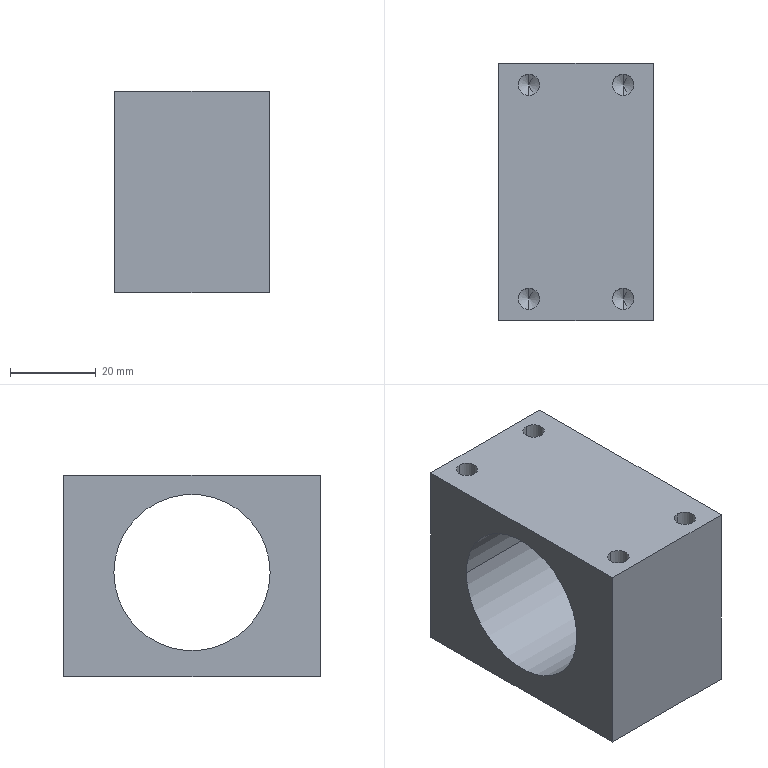Component | SolidWorks | 6G-TL06-Y-AxisMotorAssembly-2_6G-TL06.01.04-X-AxisFlangeMountingBlock-1 | 1 solid | 40 faces | box 36 x 60 x 47 mm | volume 61387 mm3 | cylinder 18 | cone 16 | plane 6 | commonest cylinder face diameters 4.2 x8 5 x8 36.5 x2
build123d program:
from build123d import *

# Parameters (mm, degrees)
SKETCH1_W             = 60
SKETCH1_H             = 36
BOSS_EXTRUDE1_DEPTH   = 47
M6_TAPPED_HOLE1_D     = 5
M6_TAPPED_HOLE1_DEPTH = 20
M6_TAPPED_HOLE1_TIP   = 1.502
M5_TAPPED_HOLE1_D     = 4.2
M5_TAPPED_HOLE1_DEPTH = 15
M5_TAPPED_HOLE1_TIP   = 1.262
SKETCH6_R             = 18.25
CUT_EXTRUDE1_DEPTH    = 67.37


with BuildPart() as part:
    # Sketch1 → Boss-Extrude1 (new body)
    with BuildSketch(Plane(origin=(0, 0, 0), x_dir=(0, 0, -1), z_dir=(1, 0, 0))):
        Rectangle(SKETCH1_W, SKETCH1_H)
    extrude(amount=BOSS_EXTRUDE1_DEPTH)

    # M6 Tapped Hole1
    with Locations(Plane(origin=(47, -3.823, -19.709), x_dir=(0, 0, 1), z_dir=(1, 0, 0))):
        with Locations((-5.291, -14.823), (-5.291, 7.177), (44.709, 7.177), (44.709, -14.823)):
            Hole(M6_TAPPED_HOLE1_D / 2, depth=M6_TAPPED_HOLE1_DEPTH)
            with Locations((0, 0, -(M6_TAPPED_HOLE1_DEPTH + M6_TAPPED_HOLE1_TIP / 2))):  # 118° drill point
                Cone(0, M6_TAPPED_HOLE1_D / 2, M6_TAPPED_HOLE1_TIP, mode=Mode.SUBTRACT)

    # M5 Tapped Hole1
    with Locations(Plane(origin=(0, -18, 0), x_dir=(-1, 0, 0), z_dir=(0, -1, 0))):
        with Locations((-40.917, -16.617), (-40.917, 16.617), (-7.683, 16.617), (-7.683, -16.617)):
            Hole(M5_TAPPED_HOLE1_D / 2, depth=M5_TAPPED_HOLE1_DEPTH)
            with Locations((0, 0, -(M5_TAPPED_HOLE1_DEPTH + M5_TAPPED_HOLE1_TIP / 2))):  # 118° drill point
                Cone(0, M5_TAPPED_HOLE1_D / 2, M5_TAPPED_HOLE1_TIP, mode=Mode.SUBTRACT)

    # Sketch6 → Cut-Extrude1 (cut, through all)
    with BuildSketch(Plane.XZ.offset(18)):
        with Locations(Location((24.3, 0, 0), (0, 0, 270))):
            Circle(SKETCH6_R)
    extrude(amount=-CUT_EXTRUDE1_DEPTH, mode=Mode.SUBTRACT)


solid = part.part

# Placed as in the assembly
solid = solid.moved(Location((-3.964, 0, -4.3), (90, 0, 90)))
STEP:
#1=CARTESIAN_POINT('',(-0.8647,-0.7185,0.7874));
#2=VERTEX_POINT('',#1);
#3=CARTESIAN_POINT('',(-0.8647,0.7185,0.7874));
#4=VERTEX_POINT('',#3);
#5=CARTESIAN_POINT('',(-0.8647,0.,0.7874));
#6=DIRECTION('',(1.,0.,-0.));
#7=DIRECTION('',(0.,1.,0.));
#8=AXIS2_PLACEMENT_3D('',#5,#6,#7);
#9=CIRCLE('',#8,0.7185);
#10=EDGE_CURVE('',#2,#4,#9,.T.);
#11=ORIENTED_EDGE('',*,*,#10,.F.);
#12=CARTESIAN_POINT('',(0.5526,-0.7185,0.7874));
#13=VERTEX_POINT('',#12);
#14=CARTESIAN_POINT('',(-0.8647,-0.7185,0.7874));
#15=DIRECTION('',(1.,0.,-0.));
#16=VECTOR('',#15,39.37);
#17=LINE('',#14,#16);
#18=EDGE_CURVE('',#2,#13,#17,.T.);
#19=ORIENTED_EDGE('',*,*,#18,.T.);
#20=CARTESIAN_POINT('',(0.5526,0.7185,0.7874));
#21=VERTEX_POINT('',#20);
#22=CARTESIAN_POINT('',(0.5526,0.,0.7874));
#23=DIRECTION('',(1.,0.,-0.));
#24=DIRECTION('',(0.,1.,0.));
#25=AXIS2_PLACEMENT_3D('',#22,#23,#24);
#26=CIRCLE('',#25,0.7185);
#27=EDGE_CURVE('',#13,#21,#26,.T.);
#28=ORIENTED_EDGE('',*,*,#27,.T.);
#29=CARTESIAN_POINT('',(-0.8647,0.7185,0.7874));
#30=DIRECTION('',(1.,0.,-0.));
#31=VECTOR('',#30,39.37);
#32=LINE('',#29,#31);
#33=EDGE_CURVE('',#4,#21,#32,.T.);
#34=ORIENTED_EDGE('',*,*,#33,.F.);
#35=EDGE_LOOP('',(#11,#19,#28,#34));
#36=FACE_OUTER_BOUND('',#35,.T.);
#37=CARTESIAN_POINT('',(-0.8647,0.,0.7874));
#38=DIRECTION('',(1.,0.,-0.));
#39=DIRECTION('',(0.,1.,0.));
#40=AXIS2_PLACEMENT_3D('',#37,#38,#39);
#41=CYLINDRICAL_SURFACE('',#40,0.7185);
#42=ADVANCED_FACE('',(#36),#41,.F.);
#43=CARTESIAN_POINT('',(-0.03795,-0.7369,1.442));
#44=VERTEX_POINT('',#43);
#45=CARTESIAN_POINT('',(-0.03795,-0.5715,1.442));
#46=VERTEX_POINT('',#45);
#47=CARTESIAN_POINT('',(-0.03795,-0.6542,1.442));
#48=DIRECTION('',(1.,0.,-0.));
#49=DIRECTION('',(0.,1.,0.));
#50=AXIS2_PLACEMENT_3D('',#47,#48,#49);
#51=CIRCLE('',#50,0.08268);
#52=EDGE_CURVE('',#44,#46,#51,.T.);
#53=ORIENTED_EDGE('',*,*,#52,.F.);
#54=CARTESIAN_POINT('',(0.5526,-0.7369,1.442));
#55=VERTEX_POINT('',#54);
#56=CARTESIAN_POINT('',(0.5526,-0.7369,1.442));
#57=DIRECTION('',(1.,0.,-0.));
#58=VECTOR('',#57,39.37);
#59=LINE('',#56,#58);
#60=EDGE_CURVE('',#44,#55,#59,.T.);
#61=ORIENTED_EDGE('',*,*,#60,.T.);
#62=CARTESIAN_POINT('',(0.5526,-0.5715,1.442));
#63=VERTEX_POINT('',#62);
#64=CARTESIAN_POINT('',(0.5526,-0.6542,1.442));
#65=DIRECTION('',(1.,0.,-0.));
#66=DIRECTION('',(0.,1.,0.));
#67=AXIS2_PLACEMENT_3D('',#64,#65,#66);
#68=CIRCLE('',#67,0.08268);
#69=EDGE_CURVE('',#55,#63,#68,.T.);
#70=ORIENTED_EDGE('',*,*,#69,.T.);
#71=CARTESIAN_POINT('',(0.5526,-0.5715,1.442));
#72=DIRECTION('',(1.,0.,-0.));
#73=VECTOR('',#72,39.37);
#74=LINE('',#71,#73);
#75=EDGE_CURVE('',#46,#63,#74,.T.);
#76=ORIENTED_EDGE('',*,*,#75,.F.);
#77=EDGE_LOOP('',(#53,#61,#70,#76));
#78=FACE_OUTER_BOUND('',#77,.T.);
#79=CARTESIAN_POINT('',(0.5526,-0.6542,1.442));
#80=DIRECTION('',(1.,0.,-0.));
#81=DIRECTION('',(0.,1.,0.));
#82=AXIS2_PLACEMENT_3D('',#79,#80,#81);
#83=CYLINDRICAL_SURFACE('',#82,0.08268);
#84=ADVANCED_FACE('',(#78),#83,.F.);
#85=CARTESIAN_POINT('',(-0.08762,-0.6542,1.442));
#86=VERTEX_POINT('',#85);
#87=CARTESIAN_POINT('',(-0.03795,-0.5715,1.442));
#88=DIRECTION('',(0.515,0.8572,0.));
#89=VECTOR('',#88,39.37);
#90=LINE('',#87,#89);
#91=EDGE_CURVE('',#86,#46,#90,.T.);
#92=ORIENTED_EDGE('',*,*,#91,.F.);
#93=CARTESIAN_POINT('',(-0.03795,-0.7369,1.442));
#94=DIRECTION('',(0.515,-0.8572,-0.));
#95=VECTOR('',#94,39.37);
#96=LINE('',#93,#95);
#97=EDGE_CURVE('',#86,#44,#96,.T.);
#98=ORIENTED_EDGE('',*,*,#97,.T.);
#99=ORIENTED_EDGE('',*,*,#52,.T.);
#100=EDGE_LOOP('',(#92,#98,#99));
#101=FACE_OUTER_BOUND('',#100,.T.);
#102=CARTESIAN_POINT('',(-0.03795,-0.6542,1.442));
#103=DIRECTION('',(1.,0.,-0.));
#104=DIRECTION('',(0.,1.,0.));
#105=AXIS2_PLACEMENT_3D('',#102,#103,#104);
#106=CONICAL_SURFACE('',#105,0.08268,1.03);
#107=ADVANCED_FACE('',(#101),#106,.F.);
#108=CARTESIAN_POINT('',(-0.03795,0.5715,1.442));
#109=VERTEX_POINT('',#108);
#110=CARTESIAN_POINT('',(-0.03795,0.7369,1.442));
#111=VERTEX_POINT('',#110);
#112=CARTESIAN_POINT('',(-0.03795,0.6542,1.442));
#113=DIRECTION('',(1.,0.,-0.));
#114=DIRECTION('',(0.,1.,0.));
#115=AXIS2_PLACEMENT_3D('',#112,#113,#114);
#116=CIRCLE('',#115,0.08268);
#117=EDGE_CURVE('',#109,#111,#116,.T.);
#118=ORIENTED_EDGE('',*,*,#117,.F.);
#119=CARTESIAN_POINT('',(0.5526,0.5715,1.442));
#120=VERTEX_POINT('',#119);
#121=CARTESIAN_POINT('',(0.5526,0.5715,1.442));
#122=DIRECTION('',(1.,0.,-0.));
#123=VECTOR('',#122,39.37);
#124=LINE('',#121,#123);
#125=EDGE_CURVE('',#109,#120,#124,.T.);
#126=ORIENTED_EDGE('',*,*,#125,.T.);
#127=CARTESIAN_POINT('',(0.5526,0.7369,1.442));
#128=VERTEX_POINT('',#127);
#129=CARTESIAN_POINT('',(0.5526,0.6542,1.442));
#130=DIRECTION('',(1.,0.,-0.));
#131=DIRECTION('',(0.,1.,0.));
#132=AXIS2_PLACEMENT_3D('',#129,#130,#131);
#133=CIRCLE('',#132,0.08268);
#134=EDGE_CURVE('',#120,#128,#133,.T.);
#135=ORIENTED_EDGE('',*,*,#134,.T.);
#136=CARTESIAN_POINT('',(0.5526,0.7369,1.442));
#137=DIRECTION('',(1.,0.,-0.));
#138=VECTOR('',#137,39.37);
#139=LINE('',#136,#138);
#140=EDGE_CURVE('',#111,#128,#139,.T.);
#141=ORIENTED_EDGE('',*,*,#140,.F.);
#142=EDGE_LOOP('',(#118,#126,#135,#141));
#143=FACE_OUTER_BOUND('',#142,.T.);
#144=CARTESIAN_POINT('',(0.5526,0.6542,1.442));
#145=DIRECTION('',(1.,0.,-0.));
#146=DIRECTION('',(0.,1.,0.));
#147=AXIS2_PLACEMENT_3D('',#144,#145,#146);
#148=CYLINDRICAL_SURFACE('',#147,0.08268);
#149=ADVANCED_FACE('',(#143),#148,.F.);
#150=CARTESIAN_POINT('',(-0.08762,0.6542,1.442));
#151=VERTEX_POINT('',#150);
#152=CARTESIAN_POINT('',(-0.03795,0.7369,1.442));
#153=DIRECTION('',(0.515,0.8572,0.));
#154=VECTOR('',#153,39.37);
#155=LINE('',#152,#154);
#156=EDGE_CURVE('',#151,#111,#155,.T.);
#157=ORIENTED_EDGE('',*,*,#156,.F.);
#158=CARTESIAN_POINT('',(-0.03795,0.5715,1.442));
#159=DIRECTION('',(0.515,-0.8572,-0.));
#160=VECTOR('',#159,39.37);
#161=LINE('',#158,#160);
#162=EDGE_CURVE('',#151,#109,#161,.T.);
#163=ORIENTED_EDGE('',*,*,#162,.T.);
#164=ORIENTED_EDGE('',*,*,#117,.T.);
#165=EDGE_LOOP('',(#157,#163,#164));
#166=FACE_OUTER_BOUND('',#165,.T.);
#167=CARTESIAN_POINT('',(-0.03795,0.6542,1.442));
#168=DIRECTION('',(1.,0.,-0.));
#169=DIRECTION('',(0.,1.,0.));
#170=AXIS2_PLACEMENT_3D('',#167,#168,#169);
#171=CONICAL_SURFACE('',#170,0.08268,1.03);
#172=ADVANCED_FACE('',(#166),#171,.F.);
#173=CARTESIAN_POINT('',(-0.03795,0.5715,0.1332));
#174=VERTEX_POINT('',#173);
#175=CARTESIAN_POINT('',(-0.03795,0.7369,0.1332));
#176=VERTEX_POINT('',#175);
#177=CARTESIAN_POINT('',(-0.03795,0.6542,0.1332));
#178=DIRECTION('',(1.,0.,-0.));
#179=DIRECTION('',(0.,1.,0.));
#180=AXIS2_PLACEMENT_3D('',#177,#178,#179);
#181=CIRCLE('',#180,0.08268);
#182=EDGE_CURVE('',#174,#176,#181,.T.);
#183=ORIENTED_EDGE('',*,*,#182,.F.);
#184=CARTESIAN_POINT('',(0.5526,0.5715,0.1332));
#185=VERTEX_POINT('',#184);
#186=CARTESIAN_POINT('',(0.5526,0.5715,0.1332));
#187=DIRECTION('',(1.,0.,-0.));
#188=VECTOR('',#187,39.37);
#189=LINE('',#186,#188);
#190=EDGE_CURVE('',#174,#185,#189,.T.);
#191=ORIENTED_EDGE('',*,*,#190,.T.);
#192=CARTESIAN_POINT('',(0.5526,0.7369,0.1332));
#193=VERTEX_POINT('',#192);
#194=CARTESIAN_POINT('',(0.5526,0.6542,0.1332));
#195=DIRECTION('',(1.,0.,-0.));
#196=DIRECTION('',(0.,1.,0.));
#197=AXIS2_PLACEMENT_3D('',#194,#195,#196);
#198=CIRCLE('',#197,0.08268);
#199=EDGE_CURVE('',#185,#193,#198,.T.);
#200=ORIENTED_EDGE('',*,*,#199,.T.);
#201=CARTESIAN_POINT('',(0.5526,0.7369,0.1332));
#202=DIRECTION('',(1.,0.,-0.));
#203=VECTOR('',#202,39.37);
#204=LINE('',#201,#203);
#205=EDGE_CURVE('',#176,#193,#204,.T.);
#206=ORIENTED_EDGE('',*,*,#205,.F.);
#207=EDGE_LOOP('',(#183,#191,#200,#206));
#208=FACE_OUTER_BOUND('',#207,.T.);
#209=CARTESIAN_POINT('',(0.5526,0.6542,0.1332));
#210=DIRECTION('',(1.,0.,-0.));
#211=DIRECTION('',(0.,1.,0.));
#212=AXIS2_PLACEMENT_3D('',#209,#210,#211);
#213=CYLINDRICAL_SURFACE('',#212,0.08268);
#214=ADVANCED_FACE('',(#208),#213,.F.);
#215=CARTESIAN_POINT('',(-0.08762,0.6542,0.1332));
#216=VERTEX_POINT('',#215);
#217=CARTESIAN_POINT('',(-0.03795,0.7369,0.1332));
#218=DIRECTION('',(0.515,0.8572,0.));
#219=VECTOR('',#218,39.37);
#220=LINE('',#217,#219);
#221=EDGE_CURVE('',#216,#176,#220,.T.);
#222=ORIENTED_EDGE('',*,*,#221,.F.);
#223=CARTESIAN_POINT('',(-0.03795,0.5715,0.1332));
#224=DIRECTION('',(0.515,-0.8572,-0.));
#225=VECTOR('',#224,39.37);
#226=LINE('',#223,#225);
#227=EDGE_CURVE('',#216,#174,#226,.T.);
#228=ORIENTED_EDGE('',*,*,#227,.T.);
#229=ORIENTED_EDGE('',*,*,#182,.T.);
#230=EDGE_LOOP('',(#222,#228,#229));
#231=FACE_OUTER_BOUND('',#230,.T.);
#232=CARTESIAN_POINT('',(-0.03795,0.6542,0.1332));
#233=DIRECTION('',(1.,0.,-0.));
#234=DIRECTION('',(0.,1.,0.));
#235=AXIS2_PLACEMENT_3D('',#232,#233,#234);
#236=CONICAL_SURFACE('',#235,0.08268,1.03);
#237=ADVANCED_FACE('',(#231),#236,.F.);
#238=CARTESIAN_POINT('',(-0.03795,-0.7369,0.1332));
#239=VERTEX_POINT('',#238);
#240=CARTESIAN_POINT('',(-0.03795,-0.5715,0.1332));
#241=VERTEX_POINT('',#240);
#242=CARTESIAN_POINT('',(-0.03795,-0.6542,0.1332));
#243=DIRECTION('',(1.,0.,-0.));
#244=DIRECTION('',(0.,1.,0.));
#245=AXIS2_PLACEMENT_3D('',#242,#243,#244);
#246=CIRCLE('',#245,0.08268);
#247=EDGE_CURVE('',#239,#241,#246,.T.);
#248=ORIENTED_EDGE('',*,*,#247,.F.);
#249=CARTESIAN_POINT('',(0.5526,-0.7369,0.1332));
#250=VERTEX_POINT('',#249);
#251=CARTESIAN_POINT('',(0.5526,-0.7369,0.1332));
#252=DIRECTION('',(1.,0.,-0.));
#253=VECTOR('',#252,39.37);
#254=LINE('',#251,#253);
#255=EDGE_CURVE('',#239,#250,#254,.T.);
#256=ORIENTED_EDGE('',*,*,#255,.T.);
#257=CARTESIAN_POINT('',(0.5526,-0.5715,0.1332));
#258=VERTEX_POINT('',#257);
#259=CARTESIAN_POINT('',(0.5526,-0.6542,0.1332));
#260=DIRECTION('',(1.,0.,-0.));
#261=DIRECTION('',(0.,1.,0.));
#262=AXIS2_PLACEMENT_3D('',#259,#260,#261);
#263=CIRCLE('',#262,0.08268);
#264=EDGE_CURVE('',#250,#258,#263,.T.);
#265=ORIENTED_EDGE('',*,*,#264,.T.);
#266=CARTESIAN_POINT('',(0.5526,-0.5715,0.1332));
#267=DIRECTION('',(1.,0.,-0.));
#268=VECTOR('',#267,39.37);
#269=LINE('',#266,#268);
#270=EDGE_CURVE('',#241,#258,#269,.T.);
#271=ORIENTED_EDGE('',*,*,#270,.F.);
#272=EDGE_LOOP('',(#248,#256,#265,#271));
#273=FACE_OUTER_BOUND('',#272,.T.);
#274=CARTESIAN_POINT('',(0.5526,-0.6542,0.1332));
#275=DIRECTION('',(1.,0.,-0.));
#276=DIRECTION('',(0.,1.,0.));
#277=AXIS2_PLACEMENT_3D('',#274,#275,#276);
#278=CYLINDRICAL_SURFACE('',#277,0.08268);
#279=ADVANCED_FACE('',(#273),#278,.F.);
#280=CARTESIAN_POINT('',(-0.08762,-0.6542,0.1332));
#281=VERTEX_POINT('',#280);
#282=CARTESIAN_POINT('',(-0.03795,-0.5715,0.1332));
#283=DIRECTION('',(0.515,0.8572,0.));
#284=VECTOR('',#283,39.37);
#285=LINE('',#282,#284);
#286=EDGE_CURVE('',#281,#241,#285,.T.);
#287=ORIENTED_EDGE('',*,*,#286,.F.);
#288=CARTESIAN_POINT('',(-0.03795,-0.7369,0.1332));
#289=DIRECTION('',(0.515,-0.8572,-0.));
#290=VECTOR('',#289,39.37);
#291=LINE('',#288,#290);
#292=EDGE_CURVE('',#281,#239,#291,.T.);
#293=ORIENTED_EDGE('',*,*,#292,.T.);
#294=ORIENTED_EDGE('',*,*,#247,.T.);
#295=EDGE_LOOP('',(#287,#293,#294));
#296=FACE_OUTER_BOUND('',#295,.T.);
#297=CARTESIAN_POINT('',(-0.03795,-0.6542,0.1332));
#298=DIRECTION('',(1.,0.,-0.));
#299=DIRECTION('',(0.,1.,0.));
#300=AXIS2_PLACEMENT_3D('',#297,#298,#299);
#301=CONICAL_SURFACE('',#300,0.08268,1.03);
#302=ADVANCED_FACE('',(#296),#301,.F.);
#303=CARTESIAN_POINT('',(-0.5891,0.8858,0.8937));
#304=VERTEX_POINT('',#303);
#305=CARTESIAN_POINT('',(-0.5891,1.083,0.8937));
#306=VERTEX_POINT('',#305);
#307=CARTESIAN_POINT('',(-0.5891,0.9843,0.8937));
#308=DIRECTION('',(0.,-0.,1.));
#309=DIRECTION('',(0.,1.,0.));
#310=AXIS2_PLACEMENT_3D('',#307,#308,#309);
#311=CIRCLE('',#310,0.09843);
#312=EDGE_CURVE('',#304,#306,#311,.T.);
#313=ORIENTED_EDGE('',*,*,#312,.F.);
#314=CARTESIAN_POINT('',(-0.5891,0.8858,1.681));
#315=VERTEX_POINT('',#314);
#316=CARTESIAN_POINT('',(-0.5891,0.8858,1.681));
#317=DIRECTION('',(0.,-0.,1.));
#318=VECTOR('',#317,39.37);
#319=LINE('',#316,#318);
#320=EDGE_CURVE('',#304,#315,#319,.T.);
#321=ORIENTED_EDGE('',*,*,#320,.T.);
#322=CARTESIAN_POINT('',(-0.5891,1.083,1.681));
#323=VERTEX_POINT('',#322);
#324=CARTESIAN_POINT('',(-0.5891,0.9843,1.681));
#325=DIRECTION('',(0.,-0.,1.));
#326=DIRECTION('',(0.,1.,0.));
#327=AXIS2_PLACEMENT_3D('',#324,#325,#326);
#328=CIRCLE('',#327,0.09843);
#329=EDGE_CURVE('',#315,#323,#328,.T.);
#330=ORIENTED_EDGE('',*,*,#329,.T.);
#331=CARTESIAN_POINT('',(-0.5891,1.083,1.681));
#332=DIRECTION('',(0.,-0.,1.));
#333=VECTOR('',#332,39.37);
#334=LINE('',#331,#333);
#335=EDGE_CURVE('',#306,#323,#334,.T.);
#336=ORIENTED_EDGE('',*,*,#335,.F.);
#337=EDGE_LOOP('',(#313,#321,#330,#336));
#338=FACE_OUTER_BOUND('',#337,.T.);
#339=CARTESIAN_POINT('',(-0.5891,0.9843,1.681));
#340=DIRECTION('',(0.,-0.,1.));
#341=DIRECTION('',(0.,1.,0.));
#342=AXIS2_PLACEMENT_3D('',#339,#340,#341);
#343=CYLINDRICAL_SURFACE('',#342,0.09843);
#344=ADVANCED_FACE('',(#338),#343,.F.);
#345=CARTESIAN_POINT('',(-0.5891,0.9843,0.8346));
#346=VERTEX_POINT('',#345);
#347=CARTESIAN_POINT('',(-0.5891,1.083,0.8937));
#348=DIRECTION('',(-0.,0.8572,0.515));
#349=VECTOR('',#348,39.37);
#350=LINE('',#347,#349);
#351=EDGE_CURVE('',#346,#306,#350,.T.);
#352=ORIENTED_EDGE('',*,*,#351,.F.);
#353=CARTESIAN_POINT('',(-0.5891,0.8858,0.8937));
#354=DIRECTION('',(-0.,-0.8572,0.515));
#355=VECTOR('',#354,39.37);
#356=LINE('',#353,#355);
#357=EDGE_CURVE('',#346,#304,#356,.T.);
#358=ORIENTED_EDGE('',*,*,#357,.T.);
#359=ORIENTED_EDGE('',*,*,#312,.T.);
#360=EDGE_LOOP('',(#352,#358,#359));
#361=FACE_OUTER_BOUND('',#360,.T.);
#362=CARTESIAN_POINT('',(-0.5891,0.9843,0.8937));
#363=DIRECTION('',(0.,-0.,1.));
#364=DIRECTION('',(0.,1.,0.));
#365=AXIS2_PLACEMENT_3D('',#362,#363,#364);
#366=CONICAL_SURFACE('',#365,0.09843,1.03);
#367=ADVANCED_FACE('',(#361),#366,.F.);
#368=CARTESIAN_POINT('',(0.277,0.8858,0.8937));
#369=VERTEX_POINT('',#368);
#370=CARTESIAN_POINT('',(0.277,1.083,0.8937));
#371=VERTEX_POINT('',#370);
#372=CARTESIAN_POINT('',(0.277,0.9843,0.8937));
#373=DIRECTION('',(0.,-0.,1.));
#374=DIRECTION('',(0.,1.,0.));
#375=AXIS2_PLACEMENT_3D('',#372,#373,#374);
#376=CIRCLE('',#375,0.09843);
#377=EDGE_CURVE('',#369,#371,#376,.T.);
#378=ORIENTED_EDGE('',*,*,#377,.F.);
#379=CARTESIAN_POINT('',(0.277,0.8858,1.681));
#380=VERTEX_POINT('',#379);
#381=CARTESIAN_POINT('',(0.277,0.8858,1.681));
#382=DIRECTION('',(0.,-0.,1.));
#383=VECTOR('',#382,39.37);
#384=LINE('',#381,#383);
#385=EDGE_CURVE('',#369,#380,#384,.T.);
#386=ORIENTED_EDGE('',*,*,#385,.T.);
#387=CARTESIAN_POINT('',(0.277,1.083,1.681));
#388=VERTEX_POINT('',#387);
#389=CARTESIAN_POINT('',(0.277,0.9843,1.681));
#390=DIRECTION('',(0.,-0.,1.));
#391=DIRECTION('',(0.,1.,0.));
#392=AXIS2_PLACEMENT_3D('',#389,#390,#391);
#393=CIRCLE('',#392,0.09843);
#394=EDGE_CURVE('',#380,#388,#393,.T.);
#395=ORIENTED_EDGE('',*,*,#394,.T.);
#396=CARTESIAN_POINT('',(0.277,1.083,1.681));
#397=DIRECTION('',(0.,-0.,1.));
#398=VECTOR('',#397,39.37);
#399=LINE('',#396,#398);
#400=EDGE_CURVE('',#371,#388,#399,.T.);
#401=ORIENTED_EDGE('',*,*,#400,.F.);
#402=EDGE_LOOP('',(#378,#386,#395,#401));
#403=FACE_OUTER_BOUND('',#402,.T.);
#404=CARTESIAN_POINT('',(0.277,0.9843,1.681));
#405=DIRECTION('',(0.,-0.,1.));
#406=DIRECTION('',(0.,1.,0.));
#407=AXIS2_PLACEMENT_3D('',#404,#405,#406);
#408=CYLINDRICAL_SURFACE('',#407,0.09843);
#409=ADVANCED_FACE('',(#403),#408,.F.);
#410=CARTESIAN_POINT('',(0.277,0.9843,0.8346));
#411=VERTEX_POINT('',#410);
#412=CARTESIAN_POINT('',(0.277,1.083,0.8937));
#413=DIRECTION('',(-0.,0.8572,0.515));
#414=VECTOR('',#413,39.37);
#415=LINE('',#412,#414);
#416=EDGE_CURVE('',#411,#371,#415,.T.);
#417=ORIENTED_EDGE('',*,*,#416,.F.);
#418=CARTESIAN_POINT('',(0.277,0.8858,0.8937));
#419=DIRECTION('',(-0.,-0.8572,0.515));
#420=VECTOR('',#419,39.37);
#421=LINE('',#418,#420);
#422=EDGE_CURVE('',#411,#369,#421,.T.);
#423=ORIENTED_EDGE('',*,*,#422,.T.);
#424=ORIENTED_EDGE('',*,*,#377,.T.);
#425=EDGE_LOOP('',(#417,#423,#424));
#426=FACE_OUTER_BOUND('',#425,.T.);
#427=CARTESIAN_POINT('',(0.277,0.9843,0.8937));
#428=DIRECTION('',(0.,-0.,1.));
#429=DIRECTION('',(0.,1.,0.));
#430=AXIS2_PLACEMENT_3D('',#427,#428,#429);
#431=CONICAL_SURFACE('',#430,0.09843,1.03);
#432=ADVANCED_FACE('',(#426),#431,.F.);
#433=CARTESIAN_POINT('',(0.277,-1.083,0.8937));
#434=VERTEX_POINT('',#433);
#435=CARTESIAN_POINT('',(0.277,-0.8858,0.8937));
#436=VERTEX_POINT('',#435);
#437=CARTESIAN_POINT('',(0.277,-0.9843,0.8937));
#438=DIRECTION('',(0.,-0.,1.));
#439=DIRECTION('',(0.,1.,0.));
#440=AXIS2_PLACEMENT_3D('',#437,#438,#439);
#441=CIRCLE('',#440,0.09843);
#442=EDGE_CURVE('',#434,#436,#441,.T.);
#443=ORIENTED_EDGE('',*,*,#442,.F.);
#444=CARTESIAN_POINT('',(0.277,-1.083,1.681));
#445=VERTEX_POINT('',#444);
#446=CARTESIAN_POINT('',(0.277,-1.083,1.681));
#447=DIRECTION('',(0.,-0.,1.));
#448=VECTOR('',#447,39.37);
#449=LINE('',#446,#448);
#450=EDGE_CURVE('',#434,#445,#449,.T.);
#451=ORIENTED_EDGE('',*,*,#450,.T.);
#452=CARTESIAN_POINT('',(0.277,-0.8858,1.681));
#453=VERTEX_POINT('',#452);
#454=CARTESIAN_POINT('',(0.277,-0.9843,1.681));
#455=DIRECTION('',(0.,-0.,1.));
#456=DIRECTION('',(0.,1.,0.));
#457=AXIS2_PLACEMENT_3D('',#454,#455,#456);
#458=CIRCLE('',#457,0.09843);
#459=EDGE_CURVE('',#445,#453,#458,.T.);
#460=ORIENTED_EDGE('',*,*,#459,.T.);
#461=CARTESIAN_POINT('',(0.277,-0.8858,1.681));
#462=DIRECTION('',(0.,-0.,1.));
#463=VECTOR('',#462,39.37);
#464=LINE('',#461,#463);
#465=EDGE_CURVE('',#436,#453,#464,.T.);
#466=ORIENTED_EDGE('',*,*,#465,.F.);
#467=EDGE_LOOP('',(#443,#451,#460,#466));
#468=FACE_OUTER_BOUND('',#467,.T.);
#469=CARTESIAN_POINT('',(0.277,-0.9843,1.681));
#470=DIRECTION('',(0.,-0.,1.));
#471=DIRECTION('',(0.,1.,0.));
#472=AXIS2_PLACEMENT_3D('',#469,#470,#471);
#473=CYLINDRICAL_SURFACE('',#472,0.09843);
#474=ADVANCED_FACE('',(#468),#473,.F.);
#475=CARTESIAN_POINT('',(0.277,-0.9843,0.8346));
#476=VERTEX_POINT('',#475);
#477=CARTESIAN_POINT('',(0.277,-0.8858,0.8937));
#478=DIRECTION('',(-0.,0.8572,0.515));
#479=VECTOR('',#478,39.37);
#480=LINE('',#477,#479);
#481=EDGE_CURVE('',#476,#436,#480,.T.);
#482=ORIENTED_EDGE('',*,*,#481,.F.);
#483=CARTESIAN_POINT('',(0.277,-1.083,0.8937));
#484=DIRECTION('',(-0.,-0.8572,0.515));
#485=VECTOR('',#484,39.37);
#486=LINE('',#483,#485);
#487=EDGE_CURVE('',#476,#434,#486,.T.);
#488=ORIENTED_EDGE('',*,*,#487,.T.);
#489=ORIENTED_EDGE('',*,*,#442,.T.);
#490=EDGE_LOOP('',(#482,#488,#489));
#491=FACE_OUTER_BOUND('',#490,.T.);
#492=CARTESIAN_POINT('',(0.277,-0.9843,0.8937));
#493=DIRECTION('',(0.,-0.,1.));
#494=DIRECTION('',(0.,1.,0.));
#495=AXIS2_PLACEMENT_3D('',#492,#493,#494);
#496=CONICAL_SURFACE('',#495,0.09843,1.03);
#497=ADVANCED_FACE('',(#491),#496,.F.);
#498=CARTESIAN_POINT('',(-0.5891,-1.083,0.8937));
#499=VERTEX_POINT('',#498);
#500=CARTESIAN_POINT('',(-0.5891,-0.8858,0.8937));
#501=VERTEX_POINT('',#500);
#502=CARTESIAN_POINT('',(-0.5891,-0.9843,0.8937));
#503=DIRECTION('',(0.,-0.,1.));
#504=DIRECTION('',(0.,1.,0.));
#505=AXIS2_PLACEMENT_3D('',#502,#503,#504);
#506=CIRCLE('',#505,0.09843);
#507=EDGE_CURVE('',#499,#501,#506,.T.);
#508=ORIENTED_EDGE('',*,*,#507,.F.);
#509=CARTESIAN_POINT('',(-0.5891,-1.083,1.681));
#510=VERTEX_POINT('',#509);
#511=CARTESIAN_POINT('',(-0.5891,-1.083,1.681));
#512=DIRECTION('',(0.,-0.,1.));
#513=VECTOR('',#512,39.37);
#514=LINE('',#511,#513);
#515=EDGE_CURVE('',#499,#510,#514,.T.);
#516=ORIENTED_EDGE('',*,*,#515,.T.);
#517=CARTESIAN_POINT('',(-0.5891,-0.8858,1.681));
#518=VERTEX_POINT('',#517);
#519=CARTESIAN_POINT('',(-0.5891,-0.9843,1.681));
#520=DIRECTION('',(0.,-0.,1.));
#521=DIRECTION('',(0.,1.,0.));
#522=AXIS2_PLACEMENT_3D('',#519,#520,#521);
#523=CIRCLE('',#522,0.09843);
#524=EDGE_CURVE('',#510,#518,#523,.T.);
#525=ORIENTED_EDGE('',*,*,#524,.T.);
#526=CARTESIAN_POINT('',(-0.5891,-0.8858,1.681));
#527=DIRECTION('',(0.,-0.,1.));
#528=VECTOR('',#527,39.37);
#529=LINE('',#526,#528);
#530=EDGE_CURVE('',#501,#518,#529,.T.);
#531=ORIENTED_EDGE('',*,*,#530,.F.);
#532=EDGE_LOOP('',(#508,#516,#525,#531));
#533=FACE_OUTER_BOUND('',#532,.T.);
#534=CARTESIAN_POINT('',(-0.5891,-0.9843,1.681));
#535=DIRECTION('',(0.,-0.,1.));
#536=DIRECTION('',(0.,1.,0.));
#537=AXIS2_PLACEMENT_3D('',#534,#535,#536);
#538=CYLINDRICAL_SURFACE('',#537,0.09843);
#539=ADVANCED_FACE('',(#533),#538,.F.);
#540=CARTESIAN_POINT('',(-0.5891,-0.9843,0.8346));
#541=VERTEX_POINT('',#540);
#542=CARTESIAN_POINT('',(-0.5891,-0.8858,0.8937));
#543=DIRECTION('',(-0.,0.8572,0.515));
#544=VECTOR('',#543,39.37);
#545=LINE('',#542,#544);
#546=EDGE_CURVE('',#541,#501,#545,.T.);
#547=ORIENTED_EDGE('',*,*,#546,.F.);
#548=CARTESIAN_POINT('',(-0.5891,-1.083,0.8937));
#549=DIRECTION('',(-0.,-0.8572,0.515));
#550=VECTOR('',#549,39.37);
#551=LINE('',#548,#550);
#552=EDGE_CURVE('',#541,#499,#551,.T.);
#553=ORIENTED_EDGE('',*,*,#552,.T.);
#554=ORIENTED_EDGE('',*,*,#507,.T.);
#555=EDGE_LOOP('',(#547,#553,#554));
#556=FACE_OUTER_BOUND('',#555,.T.);
#557=CARTESIAN_POINT('',(-0.5891,-0.9843,0.8937));
#558=DIRECTION('',(0.,-0.,1.));
#559=DIRECTION('',(0.,1.,0.));
#560=AXIS2_PLACEMENT_3D('',#557,#558,#559);
#561=CONICAL_SURFACE('',#560,0.09843,1.03);
#562=ADVANCED_FACE('',(#556),#561,.F.);
#563=CARTESIAN_POINT('',(0.5526,1.181,-0.1693));
#564=VERTEX_POINT('',#563);
#565=CARTESIAN_POINT('',(-0.8647,1.181,-0.1693));
#566=VERTEX_POINT('',#565);
#567=CARTESIAN_POINT('',(0.5526,1.181,-0.1693));
#568=DIRECTION('',(-1.,-0.,0.));
#569=VECTOR('',#568,39.37);
#570=LINE('',#567,#569);
#571=EDGE_CURVE('',#564,#566,#570,.T.);
#572=ORIENTED_EDGE('',*,*,#571,.T.);
#573=CARTESIAN_POINT('',(-0.8647,1.181,1.681));
#574=VERTEX_POINT('',#573);
#575=CARTESIAN_POINT('',(-0.8647,1.181,1.681));
#576=DIRECTION('',(-0.,0.,-1.));
#577=VECTOR('',#576,39.37);
#578=LINE('',#575,#577);
#579=EDGE_CURVE('',#574,#566,#578,.T.);
#580=ORIENTED_EDGE('',*,*,#579,.F.);
#581=CARTESIAN_POINT('',(0.5526,1.181,1.681));
#582=VERTEX_POINT('',#581);
#583=CARTESIAN_POINT('',(0.5526,1.181,1.681));
#584=DIRECTION('',(-1.,-0.,0.));
#585=VECTOR('',#584,39.37);
#586=LINE('',#583,#585);
#587=EDGE_CURVE('',#582,#574,#586,.T.);
#588=ORIENTED_EDGE('',*,*,#587,.F.);
#589=CARTESIAN_POINT('',(0.5526,1.181,1.681));
#590=DIRECTION('',(-0.,0.,-1.));
#591=VECTOR('',#590,39.37);
#592=LINE('',#589,#591);
#593=EDGE_CURVE('',#582,#564,#592,.T.);
#594=ORIENTED_EDGE('',*,*,#593,.T.);
#595=EDGE_LOOP('',(#572,#580,#588,#594));
#596=FACE_OUTER_BOUND('',#595,.T.);
#597=CARTESIAN_POINT('',(0.5526,1.181,1.681));
#598=DIRECTION('',(0.,-1.,-0.));
#599=DIRECTION('',(0.,-0.,1.));
#600=AXIS2_PLACEMENT_3D('',#597,#598,#599);
#601=PLANE('',#600);
#602=ADVANCED_FACE('',(#596),#601,.F.);
#603=CARTESIAN_POINT('',(-0.8647,0.,0.7874));
#604=DIRECTION('',(1.,0.,-0.));
#605=DIRECTION('',(0.,1.,0.));
#606=AXIS2_PLACEMENT_3D('',#603,#604,#605);
#607=CIRCLE('',#606,0.7185);
#608=EDGE_CURVE('',#4,#2,#607,.T.);
#609=ORIENTED_EDGE('',*,*,#608,.T.);
#610=ORIENTED_EDGE('',*,*,#10,.T.);
#611=EDGE_LOOP('',(#609,#610));
#612=FACE_BOUND('',#611,.T.);
#613=CARTESIAN_POINT('',(-0.8647,-1.181,-0.1693));
#614=VERTEX_POINT('',#613);
#615=CARTESIAN_POINT('',(-0.8647,-1.181,-0.1693));
#616=DIRECTION('',(0.,-1.,-0.));
#617=VECTOR('',#616,39.37);
#618=LINE('',#615,#617);
#619=EDGE_CURVE('',#566,#614,#618,.T.);
#620=ORIENTED_EDGE('',*,*,#619,.T.);
#621=CARTESIAN_POINT('',(-0.8647,-1.181,1.681));
#622=VERTEX_POINT('',#621);
#623=CARTESIAN_POINT('',(-0.8647,-1.181,1.681));
#624=DIRECTION('',(-0.,0.,-1.));
#625=VECTOR('',#624,39.37);
#626=LINE('',#623,#625);
#627=EDGE_CURVE('',#622,#614,#626,.T.);
#628=ORIENTED_EDGE('',*,*,#627,.F.);
#629=CARTESIAN_POINT('',(-0.8647,-1.181,1.681));
#630=DIRECTION('',(0.,-1.,-0.));
#631=VECTOR('',#630,39.37);
#632=LINE('',#629,#631);
#633=EDGE_CURVE('',#574,#622,#632,.T.);
#634=ORIENTED_EDGE('',*,*,#633,.F.);
#635=ORIENTED_EDGE('',*,*,#579,.T.);
#636=EDGE_LOOP('',(#620,#628,#634,#635));
#637=FACE_OUTER_BOUND('',#636,.T.);
#638=CARTESIAN_POINT('',(-0.8647,-1.181,1.681));
#639=DIRECTION('',(1.,0.,-0.));
#640=DIRECTION('',(-0.,1.,0.));
#641=AXIS2_PLACEMENT_3D('',#638,#639,#640);
#642=PLANE('',#641);
#643=ADVANCED_FACE('',(#612,#637),#642,.F.);
#644=CARTESIAN_POINT('',(0.5526,-1.181,-0.1693));
#645=VERTEX_POINT('',#644);
#646=CARTESIAN_POINT('',(0.5526,-1.181,-0.1693));
#647=DIRECTION('',(1.,0.,-0.));
#648=VECTOR('',#647,39.37);
#649=LINE('',#646,#648);
#650=EDGE_CURVE('',#614,#645,#649,.T.);
#651=ORIENTED_EDGE('',*,*,#650,.T.);
#652=CARTESIAN_POINT('',(0.5526,-1.181,1.681));
#653=VERTEX_POINT('',#652);
#654=CARTESIAN_POINT('',(0.5526,-1.181,1.681));
#655=DIRECTION('',(-0.,0.,-1.));
#656=VECTOR('',#655,39.37);
#657=LINE('',#654,#656);
#658=EDGE_CURVE('',#653,#645,#657,.T.);
#659=ORIENTED_EDGE('',*,*,#658,.F.);
#660=CARTESIAN_POINT('',(0.5526,-1.181,1.681));
#661=DIRECTION('',(1.,0.,-0.));
#662=VECTOR('',#661,39.37);
#663=LINE('',#660,#662);
#664=EDGE_CURVE('',#622,#653,#663,.T.);
#665=ORIENTED_EDGE('',*,*,#664,.F.);
#666=ORIENTED_EDGE('',*,*,#627,.T.);
#667=EDGE_LOOP('',(#651,#659,#665,#666));
#668=FACE_OUTER_BOUND('',#667,.T.);
#669=CARTESIAN_POINT('',(0.5526,-1.181,1.681));
#670=DIRECTION('',(-0.,1.,0.));
#671=DIRECTION('',(-0.,0.,-1.));
#672=AXIS2_PLACEMENT_3D('',#669,#670,#671);
#673=PLANE('',#672);
#674=ADVANCED_FACE('',(#668),#673,.F.);
#675=CARTESIAN_POINT('',(0.5526,0.,0.7874));
#676=DIRECTION('',(1.,0.,-0.));
#677=DIRECTION('',(0.,1.,0.));
#678=AXIS2_PLACEMENT_3D('',#675,#676,#677);
#679=CIRCLE('',#678,0.7185);
#680=EDGE_CURVE('',#21,#13,#679,.T.);
#681=ORIENTED_EDGE('',*,*,#680,.F.);
#682=ORIENTED_EDGE('',*,*,#27,.F.);
#683=EDGE_LOOP('',(#681,#682));
#684=FACE_BOUND('',#683,.T.);
#685=CARTESIAN_POINT('',(0.5526,-0.6542,1.442));
#686=DIRECTION('',(1.,0.,-0.));
#687=DIRECTION('',(0.,1.,0.));
#688=AXIS2_PLACEMENT_3D('',#685,#686,#687);
#689=CIRCLE('',#688,0.08268);
#690=EDGE_CURVE('',#63,#55,#689,.T.);
#691=ORIENTED_EDGE('',*,*,#690,.F.);
#692=ORIENTED_EDGE('',*,*,#69,.F.);
#693=EDGE_LOOP('',(#691,#692));
#694=FACE_BOUND('',#693,.T.);
#695=CARTESIAN_POINT('',(0.5526,0.6542,1.442));
#696=DIRECTION('',(1.,0.,-0.));
#697=DIRECTION('',(0.,1.,0.));
#698=AXIS2_PLACEMENT_3D('',#695,#696,#697);
#699=CIRCLE('',#698,0.08268);
#700=EDGE_CURVE('',#128,#120,#699,.T.);
#701=ORIENTED_EDGE('',*,*,#700,.F.);
#702=ORIENTED_EDGE('',*,*,#134,.F.);
#703=EDGE_LOOP('',(#701,#702));
#704=FACE_BOUND('',#703,.T.);
#705=CARTESIAN_POINT('',(0.5526,0.6542,0.1332));
#706=DIRECTION('',(1.,0.,-0.));
#707=DIRECTION('',(0.,1.,0.));
#708=AXIS2_PLACEMENT_3D('',#705,#706,#707);
#709=CIRCLE('',#708,0.08268);
#710=EDGE_CURVE('',#193,#185,#709,.T.);
#711=ORIENTED_EDGE('',*,*,#710,.F.);
#712=ORIENTED_EDGE('',*,*,#199,.F.);
#713=EDGE_LOOP('',(#711,#712));
#714=FACE_BOUND('',#713,.T.);
#715=CARTESIAN_POINT('',(0.5526,-0.6542,0.1332));
#716=DIRECTION('',(1.,0.,-0.));
#717=DIRECTION('',(0.,1.,0.));
#718=AXIS2_PLACEMENT_3D('',#715,#716,#717);
#719=CIRCLE('',#718,0.08268);
#720=EDGE_CURVE('',#258,#250,#719,.T.);
#721=ORIENTED_EDGE('',*,*,#720,.F.);
#722=ORIENTED_EDGE('',*,*,#264,.F.);
#723=EDGE_LOOP('',(#721,#722));
#724=FACE_BOUND('',#723,.T.);
#725=CARTESIAN_POINT('',(0.5526,-1.181,-0.1693));
#726=DIRECTION('',(-0.,1.,0.));
#727=VECTOR('',#726,39.37);
#728=LINE('',#725,#727);
#729=EDGE_CURVE('',#645,#564,#728,.T.);
#730=ORIENTED_EDGE('',*,*,#729,.T.);
#731=ORIENTED_EDGE('',*,*,#593,.F.);
#732=CARTESIAN_POINT('',(0.5526,-1.181,1.681));
#733=DIRECTION('',(-0.,1.,0.));
#734=VECTOR('',#733,39.37);
#735=LINE('',#732,#734);
#736=EDGE_CURVE('',#653,#582,#735,.T.);
#737=ORIENTED_EDGE('',*,*,#736,.F.);
#738=ORIENTED_EDGE('',*,*,#658,.T.);
#739=EDGE_LOOP('',(#730,#731,#737,#738));
#740=FACE_OUTER_BOUND('',#739,.T.);
#741=CARTESIAN_POINT('',(0.5526,-1.181,1.681));
#742=DIRECTION('',(-1.,-0.,0.));
#743=DIRECTION('',(0.,-1.,-0.));
#744=AXIS2_PLACEMENT_3D('',#741,#742,#743);
#745=PLANE('',#744);
#746=ADVANCED_FACE('',(#684,#694,#704,#714,#724,#740),#745,.F.);
#747=CARTESIAN_POINT('',(-0.5891,0.9843,1.681));
#748=DIRECTION('',(0.,-0.,1.));
#749=DIRECTION('',(0.,1.,0.));
#750=AXIS2_PLACEMENT_3D('',#747,#748,#749);
#751=CIRCLE('',#750,0.09843);
#752=EDGE_CURVE('',#323,#315,#751,.T.);
#753=ORIENTED_EDGE('',*,*,#752,.F.);
#754=ORIENTED_EDGE('',*,*,#329,.F.);
#755=EDGE_LOOP('',(#753,#754));
#756=FACE_BOUND('',#755,.T.);
#757=CARTESIAN_POINT('',(0.277,0.9843,1.681));
#758=DIRECTION('',(0.,-0.,1.));
#759=DIRECTION('',(0.,1.,0.));
#760=AXIS2_PLACEMENT_3D('',#757,#758,#759);
#761=CIRCLE('',#760,0.09843);
#762=EDGE_CURVE('',#388,#380,#761,.T.);
#763=ORIENTED_EDGE('',*,*,#762,.F.);
#764=ORIENTED_EDGE('',*,*,#394,.F.);
#765=EDGE_LOOP('',(#763,#764));
#766=FACE_BOUND('',#765,.T.);
#767=CARTESIAN_POINT('',(0.277,-0.9843,1.681));
#768=DIRECTION('',(0.,-0.,1.));
#769=DIRECTION('',(0.,1.,0.));
#770=AXIS2_PLACEMENT_3D('',#767,#768,#769);
#771=CIRCLE('',#770,0.09843);
#772=EDGE_CURVE('',#453,#445,#771,.T.);
#773=ORIENTED_EDGE('',*,*,#772,.F.);
#774=ORIENTED_EDGE('',*,*,#459,.F.);
#775=EDGE_LOOP('',(#773,#774));
#776=FACE_BOUND('',#775,.T.);
#777=CARTESIAN_POINT('',(-0.5891,-0.9843,1.681));
#778=DIRECTION('',(0.,-0.,1.));
#779=DIRECTION('',(0.,1.,0.));
#780=AXIS2_PLACEMENT_3D('',#777,#778,#779);
#781=CIRCLE('',#780,0.09843);
#782=EDGE_CURVE('',#518,#510,#781,.T.);
#783=ORIENTED_EDGE('',*,*,#782,.F.);
#784=ORIENTED_EDGE('',*,*,#524,.F.);
#785=EDGE_LOOP('',(#783,#784));
#786=FACE_BOUND('',#785,.T.);
#787=ORIENTED_EDGE('',*,*,#587,.T.);
#788=ORIENTED_EDGE('',*,*,#633,.T.);
#789=ORIENTED_EDGE('',*,*,#664,.T.);
#790=ORIENTED_EDGE('',*,*,#736,.T.);
#791=EDGE_LOOP('',(#787,#788,#789,#790));
#792=FACE_OUTER_BOUND('',#791,.T.);
#793=CARTESIAN_POINT('',(-0.1561,-0.,1.681));
#794=DIRECTION('',(-0.,0.,-1.));
#795=DIRECTION('',(0.,-1.,-0.));
#796=AXIS2_PLACEMENT_3D('',#793,#794,#795);
#797=PLANE('',#796);
#798=ADVANCED_FACE('',(#756,#766,#776,#786,#792),#797,.F.);
#799=ORIENTED_EDGE('',*,*,#571,.F.);
#800=ORIENTED_EDGE('',*,*,#729,.F.);
#801=ORIENTED_EDGE('',*,*,#650,.F.);
#802=ORIENTED_EDGE('',*,*,#619,.F.);
#803=EDGE_LOOP('',(#799,#800,#801,#802));
#804=FACE_OUTER_BOUND('',#803,.T.);
#805=CARTESIAN_POINT('',(-0.1561,0.,-0.1693));
#806=DIRECTION('',(-0.,0.,-1.));
#807=DIRECTION('',(0.,-1.,-0.));
#808=AXIS2_PLACEMENT_3D('',#805,#806,#807);
#809=PLANE('',#808);
#810=ADVANCED_FACE('',(#804),#809,.T.);
#811=ORIENTED_EDGE('',*,*,#552,.F.);
#812=ORIENTED_EDGE('',*,*,#546,.T.);
#813=CARTESIAN_POINT('',(-0.5891,-0.9843,0.8937));
#814=DIRECTION('',(0.,-0.,1.));
#815=DIRECTION('',(0.,1.,0.));
#816=AXIS2_PLACEMENT_3D('',#813,#814,#815);
#817=CIRCLE('',#816,0.09843);
#818=EDGE_CURVE('',#501,#499,#817,.T.);
#819=ORIENTED_EDGE('',*,*,#818,.T.);
#820=EDGE_LOOP('',(#811,#812,#819));
#821=FACE_OUTER_BOUND('',#820,.T.);
#822=CARTESIAN_POINT('',(-0.5891,-0.9843,0.8937));
#823=DIRECTION('',(0.,-0.,1.));
#824=DIRECTION('',(0.,1.,0.));
#825=AXIS2_PLACEMENT_3D('',#822,#823,#824);
#826=CONICAL_SURFACE('',#825,0.09843,1.03);
#827=ADVANCED_FACE('',(#821),#826,.F.);
#828=ORIENTED_EDGE('',*,*,#515,.F.);
#829=ORIENTED_EDGE('',*,*,#818,.F.);
#830=ORIENTED_EDGE('',*,*,#530,.T.);
#831=ORIENTED_EDGE('',*,*,#782,.T.);
#832=EDGE_LOOP('',(#828,#829,#830,#831));
#833=FACE_OUTER_BOUND('',#832,.T.);
#834=CARTESIAN_POINT('',(-0.5891,-0.9843,1.681));
#835=DIRECTION('',(0.,-0.,1.));
#836=DIRECTION('',(0.,1.,0.));
#837=AXIS2_PLACEMENT_3D('',#834,#835,#836);
#838=CYLINDRICAL_SURFACE('',#837,0.09843);
#839=ADVANCED_FACE('',(#833),#838,.F.);
#840=ORIENTED_EDGE('',*,*,#487,.F.);
#841=ORIENTED_EDGE('',*,*,#481,.T.);
#842=CARTESIAN_POINT('',(0.277,-0.9843,0.8937));
#843=DIRECTION('',(0.,-0.,1.));
#844=DIRECTION('',(0.,1.,0.));
#845=AXIS2_PLACEMENT_3D('',#842,#843,#844);
#846=CIRCLE('',#845,0.09843);
#847=EDGE_CURVE('',#436,#434,#846,.T.);
#848=ORIENTED_EDGE('',*,*,#847,.T.);
#849=EDGE_LOOP('',(#840,#841,#848));
#850=FACE_OUTER_BOUND('',#849,.T.);
#851=CARTESIAN_POINT('',(0.277,-0.9843,0.8937));
#852=DIRECTION('',(0.,-0.,1.));
#853=DIRECTION('',(0.,1.,0.));
#854=AXIS2_PLACEMENT_3D('',#851,#852,#853);
#855=CONICAL_SURFACE('',#854,0.09843,1.03);
#856=ADVANCED_FACE('',(#850),#855,.F.);
#857=ORIENTED_EDGE('',*,*,#450,.F.);
#858=ORIENTED_EDGE('',*,*,#847,.F.);
#859=ORIENTED_EDGE('',*,*,#465,.T.);
#860=ORIENTED_EDGE('',*,*,#772,.T.);
#861=EDGE_LOOP('',(#857,#858,#859,#860));
#862=FACE_OUTER_BOUND('',#861,.T.);
#863=CARTESIAN_POINT('',(0.277,-0.9843,1.681));
#864=DIRECTION('',(0.,-0.,1.));
#865=DIRECTION('',(0.,1.,0.));
#866=AXIS2_PLACEMENT_3D('',#863,#864,#865);
#867=CYLINDRICAL_SURFACE('',#866,0.09843);
#868=ADVANCED_FACE('',(#862),#867,.F.);
#869=ORIENTED_EDGE('',*,*,#422,.F.);
#870=ORIENTED_EDGE('',*,*,#416,.T.);
#871=CARTESIAN_POINT('',(0.277,0.9843,0.8937));
#872=DIRECTION('',(0.,-0.,1.));
#873=DIRECTION('',(0.,1.,0.));
#874=AXIS2_PLACEMENT_3D('',#871,#872,#873);
#875=CIRCLE('',#874,0.09843);
#876=EDGE_CURVE('',#371,#369,#875,.T.);
#877=ORIENTED_EDGE('',*,*,#876,.T.);
#878=EDGE_LOOP('',(#869,#870,#877));
#879=FACE_OUTER_BOUND('',#878,.T.);
#880=CARTESIAN_POINT('',(0.277,0.9843,0.8937));
#881=DIRECTION('',(0.,-0.,1.));
#882=DIRECTION('',(0.,1.,0.));
#883=AXIS2_PLACEMENT_3D('',#880,#881,#882);
#884=CONICAL_SURFACE('',#883,0.09843,1.03);
#885=ADVANCED_FACE('',(#879),#884,.F.);
#886=ORIENTED_EDGE('',*,*,#385,.F.);
#887=ORIENTED_EDGE('',*,*,#876,.F.);
#888=ORIENTED_EDGE('',*,*,#400,.T.);
#889=ORIENTED_EDGE('',*,*,#762,.T.);
#890=EDGE_LOOP('',(#886,#887,#888,#889));
#891=FACE_OUTER_BOUND('',#890,.T.);
#892=CARTESIAN_POINT('',(0.277,0.9843,1.681));
#893=DIRECTION('',(0.,-0.,1.));
#894=DIRECTION('',(0.,1.,0.));
#895=AXIS2_PLACEMENT_3D('',#892,#893,#894);
#896=CYLINDRICAL_SURFACE('',#895,0.09843);
#897=ADVANCED_FACE('',(#891),#896,.F.);
#898=ORIENTED_EDGE('',*,*,#357,.F.);
#899=ORIENTED_EDGE('',*,*,#351,.T.);
#900=CARTESIAN_POINT('',(-0.5891,0.9843,0.8937));
#901=DIRECTION('',(0.,-0.,1.));
#902=DIRECTION('',(0.,1.,0.));
#903=AXIS2_PLACEMENT_3D('',#900,#901,#902);
#904=CIRCLE('',#903,0.09843);
#905=EDGE_CURVE('',#306,#304,#904,.T.);
#906=ORIENTED_EDGE('',*,*,#905,.T.);
#907=EDGE_LOOP('',(#898,#899,#906));
#908=FACE_OUTER_BOUND('',#907,.T.);
#909=CARTESIAN_POINT('',(-0.5891,0.9843,0.8937));
#910=DIRECTION('',(0.,-0.,1.));
#911=DIRECTION('',(0.,1.,0.));
#912=AXIS2_PLACEMENT_3D('',#909,#910,#911);
#913=CONICAL_SURFACE('',#912,0.09843,1.03);
#914=ADVANCED_FACE('',(#908),#913,.F.);
#915=ORIENTED_EDGE('',*,*,#320,.F.);
#916=ORIENTED_EDGE('',*,*,#905,.F.);
#917=ORIENTED_EDGE('',*,*,#335,.T.);
#918=ORIENTED_EDGE('',*,*,#752,.T.);
#919=EDGE_LOOP('',(#915,#916,#917,#918));
#920=FACE_OUTER_BOUND('',#919,.T.);
#921=CARTESIAN_POINT('',(-0.5891,0.9843,1.681));
#922=DIRECTION('',(0.,-0.,1.));
#923=DIRECTION('',(0.,1.,0.));
#924=AXIS2_PLACEMENT_3D('',#921,#922,#923);
#925=CYLINDRICAL_SURFACE('',#924,0.09843);
#926=ADVANCED_FACE('',(#920),#925,.F.);
#927=ORIENTED_EDGE('',*,*,#292,.F.);
#928=ORIENTED_EDGE('',*,*,#286,.T.);
#929=CARTESIAN_POINT('',(-0.03795,-0.6542,0.1332));
#930=DIRECTION('',(1.,0.,-0.));
#931=DIRECTION('',(0.,1.,0.));
#932=AXIS2_PLACEMENT_3D('',#929,#930,#931);
#933=CIRCLE('',#932,0.08268);
#934=EDGE_CURVE('',#241,#239,#933,.T.);
#935=ORIENTED_EDGE('',*,*,#934,.T.);
#936=EDGE_LOOP('',(#927,#928,#935));
#937=FACE_OUTER_BOUND('',#936,.T.);
#938=CARTESIAN_POINT('',(-0.03795,-0.6542,0.1332));
#939=DIRECTION('',(1.,0.,-0.));
#940=DIRECTION('',(0.,1.,0.));
#941=AXIS2_PLACEMENT_3D('',#938,#939,#940);
#942=CONICAL_SURFACE('',#941,0.08268,1.03);
#943=ADVANCED_FACE('',(#937),#942,.F.);
#944=ORIENTED_EDGE('',*,*,#255,.F.);
#945=ORIENTED_EDGE('',*,*,#934,.F.);
#946=ORIENTED_EDGE('',*,*,#270,.T.);
#947=ORIENTED_EDGE('',*,*,#720,.T.);
#948=EDGE_LOOP('',(#944,#945,#946,#947));
#949=FACE_OUTER_BOUND('',#948,.T.);
#950=CARTESIAN_POINT('',(0.5526,-0.6542,0.1332));
#951=DIRECTION('',(1.,0.,-0.));
#952=DIRECTION('',(0.,1.,0.));
#953=AXIS2_PLACEMENT_3D('',#950,#951,#952);
#954=CYLINDRICAL_SURFACE('',#953,0.08268);
#955=ADVANCED_FACE('',(#949),#954,.F.);
#956=ORIENTED_EDGE('',*,*,#227,.F.);
#957=ORIENTED_EDGE('',*,*,#221,.T.);
#958=CARTESIAN_POINT('',(-0.03795,0.6542,0.1332));
#959=DIRECTION('',(1.,0.,-0.));
#960=DIRECTION('',(0.,1.,0.));
#961=AXIS2_PLACEMENT_3D('',#958,#959,#960);
#962=CIRCLE('',#961,0.08268);
#963=EDGE_CURVE('',#176,#174,#962,.T.);
#964=ORIENTED_EDGE('',*,*,#963,.T.);
#965=EDGE_LOOP('',(#956,#957,#964));
#966=FACE_OUTER_BOUND('',#965,.T.);
#967=CARTESIAN_POINT('',(-0.03795,0.6542,0.1332));
#968=DIRECTION('',(1.,0.,-0.));
#969=DIRECTION('',(0.,1.,0.));
#970=AXIS2_PLACEMENT_3D('',#967,#968,#969);
#971=CONICAL_SURFACE('',#970,0.08268,1.03);
#972=ADVANCED_FACE('',(#966),#971,.F.);
#973=ORIENTED_EDGE('',*,*,#190,.F.);
#974=ORIENTED_EDGE('',*,*,#963,.F.);
#975=ORIENTED_EDGE('',*,*,#205,.T.);
#976=ORIENTED_EDGE('',*,*,#710,.T.);
#977=EDGE_LOOP('',(#973,#974,#975,#976));
#978=FACE_OUTER_BOUND('',#977,.T.);
#979=CARTESIAN_POINT('',(0.5526,0.6542,0.1332));
#980=DIRECTION('',(1.,0.,-0.));
#981=DIRECTION('',(0.,1.,0.));
#982=AXIS2_PLACEMENT_3D('',#979,#980,#981);
#983=CYLINDRICAL_SURFACE('',#982,0.08268);
#984=ADVANCED_FACE('',(#978),#983,.F.);
#985=ORIENTED_EDGE('',*,*,#162,.F.);
#986=ORIENTED_EDGE('',*,*,#156,.T.);
#987=CARTESIAN_POINT('',(-0.03795,0.6542,1.442));
#988=DIRECTION('',(1.,0.,-0.));
#989=DIRECTION('',(0.,1.,0.));
#990=AXIS2_PLACEMENT_3D('',#987,#988,#989);
#991=CIRCLE('',#990,0.08268);
#992=EDGE_CURVE('',#111,#109,#991,.T.);
#993=ORIENTED_EDGE('',*,*,#992,.T.);
#994=EDGE_LOOP('',(#985,#986,#993));
#995=FACE_OUTER_BOUND('',#994,.T.);
#996=CARTESIAN_POINT('',(-0.03795,0.6542,1.442));
#997=DIRECTION('',(1.,0.,-0.));
#998=DIRECTION('',(0.,1.,0.));
#999=AXIS2_PLACEMENT_3D('',#996,#997,#998);
#1000=CONICAL_SURFACE('',#999,0.08268,1.03);
#1001=ADVANCED_FACE('',(#995),#1000,.F.);
#1002=ORIENTED_EDGE('',*,*,#125,.F.);
#1003=ORIENTED_EDGE('',*,*,#992,.F.);
#1004=ORIENTED_EDGE('',*,*,#140,.T.);
#1005=ORIENTED_EDGE('',*,*,#700,.T.);
#1006=EDGE_LOOP('',(#1002,#1003,#1004,#1005));
#1007=FACE_OUTER_BOUND('',#1006,.T.);
#1008=CARTESIAN_POINT('',(0.5526,0.6542,1.442));
#1009=DIRECTION('',(1.,0.,-0.));
#1010=DIRECTION('',(0.,1.,0.));
#1011=AXIS2_PLACEMENT_3D('',#1008,#1009,#1010);
#1012=CYLINDRICAL_SURFACE('',#1011,0.08268);
#1013=ADVANCED_FACE('',(#1007),#1012,.F.);
#1014=ORIENTED_EDGE('',*,*,#97,.F.);
#1015=ORIENTED_EDGE('',*,*,#91,.T.);
#1016=CARTESIAN_POINT('',(-0.03795,-0.6542,1.442));
#1017=DIRECTION('',(1.,0.,-0.));
#1018=DIRECTION('',(0.,1.,0.));
#1019=AXIS2_PLACEMENT_3D('',#1016,#1017,#1018);
#1020=CIRCLE('',#1019,0.08268);
#1021=EDGE_CURVE('',#46,#44,#1020,.T.);
#1022=ORIENTED_EDGE('',*,*,#1021,.T.);
#1023=EDGE_LOOP('',(#1014,#1015,#1022));
#1024=FACE_OUTER_BOUND('',#1023,.T.);
#1025=CARTESIAN_POINT('',(-0.03795,-0.6542,1.442));
#1026=DIRECTION('',(1.,0.,-0.));
#1027=DIRECTION('',(0.,1.,0.));
#1028=AXIS2_PLACEMENT_3D('',#1025,#1026,#1027);
#1029=CONICAL_SURFACE('',#1028,0.08268,1.03);
#1030=ADVANCED_FACE('',(#1024),#1029,.F.);
#1031=ORIENTED_EDGE('',*,*,#60,.F.);
#1032=ORIENTED_EDGE('',*,*,#1021,.F.);
#1033=ORIENTED_EDGE('',*,*,#75,.T.);
#1034=ORIENTED_EDGE('',*,*,#690,.T.);
#1035=EDGE_LOOP('',(#1031,#1032,#1033,#1034));
#1036=FACE_OUTER_BOUND('',#1035,.T.);
#1037=CARTESIAN_POINT('',(0.5526,-0.6542,1.442));
#1038=DIRECTION('',(1.,0.,-0.));
#1039=DIRECTION('',(0.,1.,0.));
#1040=AXIS2_PLACEMENT_3D('',#1037,#1038,#1039);
#1041=CYLINDRICAL_SURFACE('',#1040,0.08268);
#1042=ADVANCED_FACE('',(#1036),#1041,.F.);
#1043=ORIENTED_EDGE('',*,*,#18,.F.);
#1044=ORIENTED_EDGE('',*,*,#608,.F.);
#1045=ORIENTED_EDGE('',*,*,#33,.T.);
#1046=ORIENTED_EDGE('',*,*,#680,.T.);
#1047=EDGE_LOOP('',(#1043,#1044,#1045,#1046));
#1048=FACE_OUTER_BOUND('',#1047,.T.);
#1049=CARTESIAN_POINT('',(-0.8647,0.,0.7874));
#1050=DIRECTION('',(1.,0.,-0.));
#1051=DIRECTION('',(0.,1.,0.));
#1052=AXIS2_PLACEMENT_3D('',#1049,#1050,#1051);
#1053=CYLINDRICAL_SURFACE('',#1052,0.7185);
#1054=ADVANCED_FACE('',(#1048),#1053,.F.);
#1055=CLOSED_SHELL('',(#42,#84,#107,#149,#172,#214,#237,#279,#302,#344,#367,#409,#432,#474,#497,#539,#562,#602,#643,#674,#746,#798,#810,#827,#839,#856,#868,#885,#897,#914,#926,#943,#955,#972,#984,#1001,#1013,#1030,#1042,#1054));
#1056=MANIFOLD_SOLID_BREP('',#1055);
#1057=CARTESIAN_POINT('',(0.,0.,0.));
#1058=DIRECTION('',(0.,0.,1.));
#1059=DIRECTION('',(1.,0.,0.));
#1060=AXIS2_PLACEMENT_3D('',#1057,#1058,#1059);
#1061=(LENGTH_UNIT()NAMED_UNIT(*)SI_UNIT($,.METRE.));
#1062=LENGTH_MEASURE_WITH_UNIT(LENGTH_MEASURE(0.0254),#1061);
#1063=DIMENSIONAL_EXPONENTS(1.,0.,0.,0.,0.,0.,0.);
#1064=(CONVERSION_BASED_UNIT('',#1062)LENGTH_UNIT()NAMED_UNIT(#1063));
#1065=UNCERTAINTY_MEASURE_WITH_UNIT(LENGTH_MEASURE(0.00001),#1064,'','');
#1066=(NAMED_UNIT(*)PLANE_ANGLE_UNIT()SI_UNIT($,.RADIAN.));
#1067=(NAMED_UNIT(*)SI_UNIT($,.STERADIAN.)SOLID_ANGLE_UNIT());
#1068=(GEOMETRIC_REPRESENTATION_CONTEXT(3)GLOBAL_UNCERTAINTY_ASSIGNED_CONTEXT((#1065))GLOBAL_UNIT_ASSIGNED_CONTEXT((#1064,#1066,#1067))REPRESENTATION_CONTEXT('',''));
#1069=ADVANCED_BREP_SHAPE_REPRESENTATION('',(#1056,#1060),#1068);
#1070=COLOUR_RGB('',0.7922,0.8196,0.9333);
#1071=FILL_AREA_STYLE_COLOUR('',#1070);
#1072=FILL_AREA_STYLE('',(#1071));
#1073=SURFACE_STYLE_FILL_AREA(#1072);
#1074=SURFACE_SIDE_STYLE('',(#1073));
#1075=SURFACE_STYLE_USAGE(.BOTH.,#1074);
#1076=PRESENTATION_STYLE_ASSIGNMENT((#1075));
#1077=STYLED_ITEM('',(#1076),#1056);
#1078=(LENGTH_UNIT()NAMED_UNIT(*)SI_UNIT($,.METRE.));
#1079=LENGTH_MEASURE_WITH_UNIT(LENGTH_MEASURE(0.0254),#1078);
#1080=DIMENSIONAL_EXPONENTS(1.,0.,0.,0.,0.,0.,0.);
#1081=(CONVERSION_BASED_UNIT('',#1079)LENGTH_UNIT()NAMED_UNIT(#1080));
#1082=UNCERTAINTY_MEASURE_WITH_UNIT(LENGTH_MEASURE(0.00001),#1081,'','');
#1083=(NAMED_UNIT(*)PLANE_ANGLE_UNIT()SI_UNIT($,.RADIAN.));
#1084=(NAMED_UNIT(*)SI_UNIT($,.STERADIAN.)SOLID_ANGLE_UNIT());
#1085=(GEOMETRIC_REPRESENTATION_CONTEXT(3)GLOBAL_UNCERTAINTY_ASSIGNED_CONTEXT((#1082))GLOBAL_UNIT_ASSIGNED_CONTEXT((#1081,#1083,#1084))REPRESENTATION_CONTEXT('',''));
#1086=MECHANICAL_DESIGN_GEOMETRIC_PRESENTATION_REPRESENTATION('',(#1077),#1085);
#1087=PRESENTATION_LAYER_ASSIGNMENT('','',(#1077));